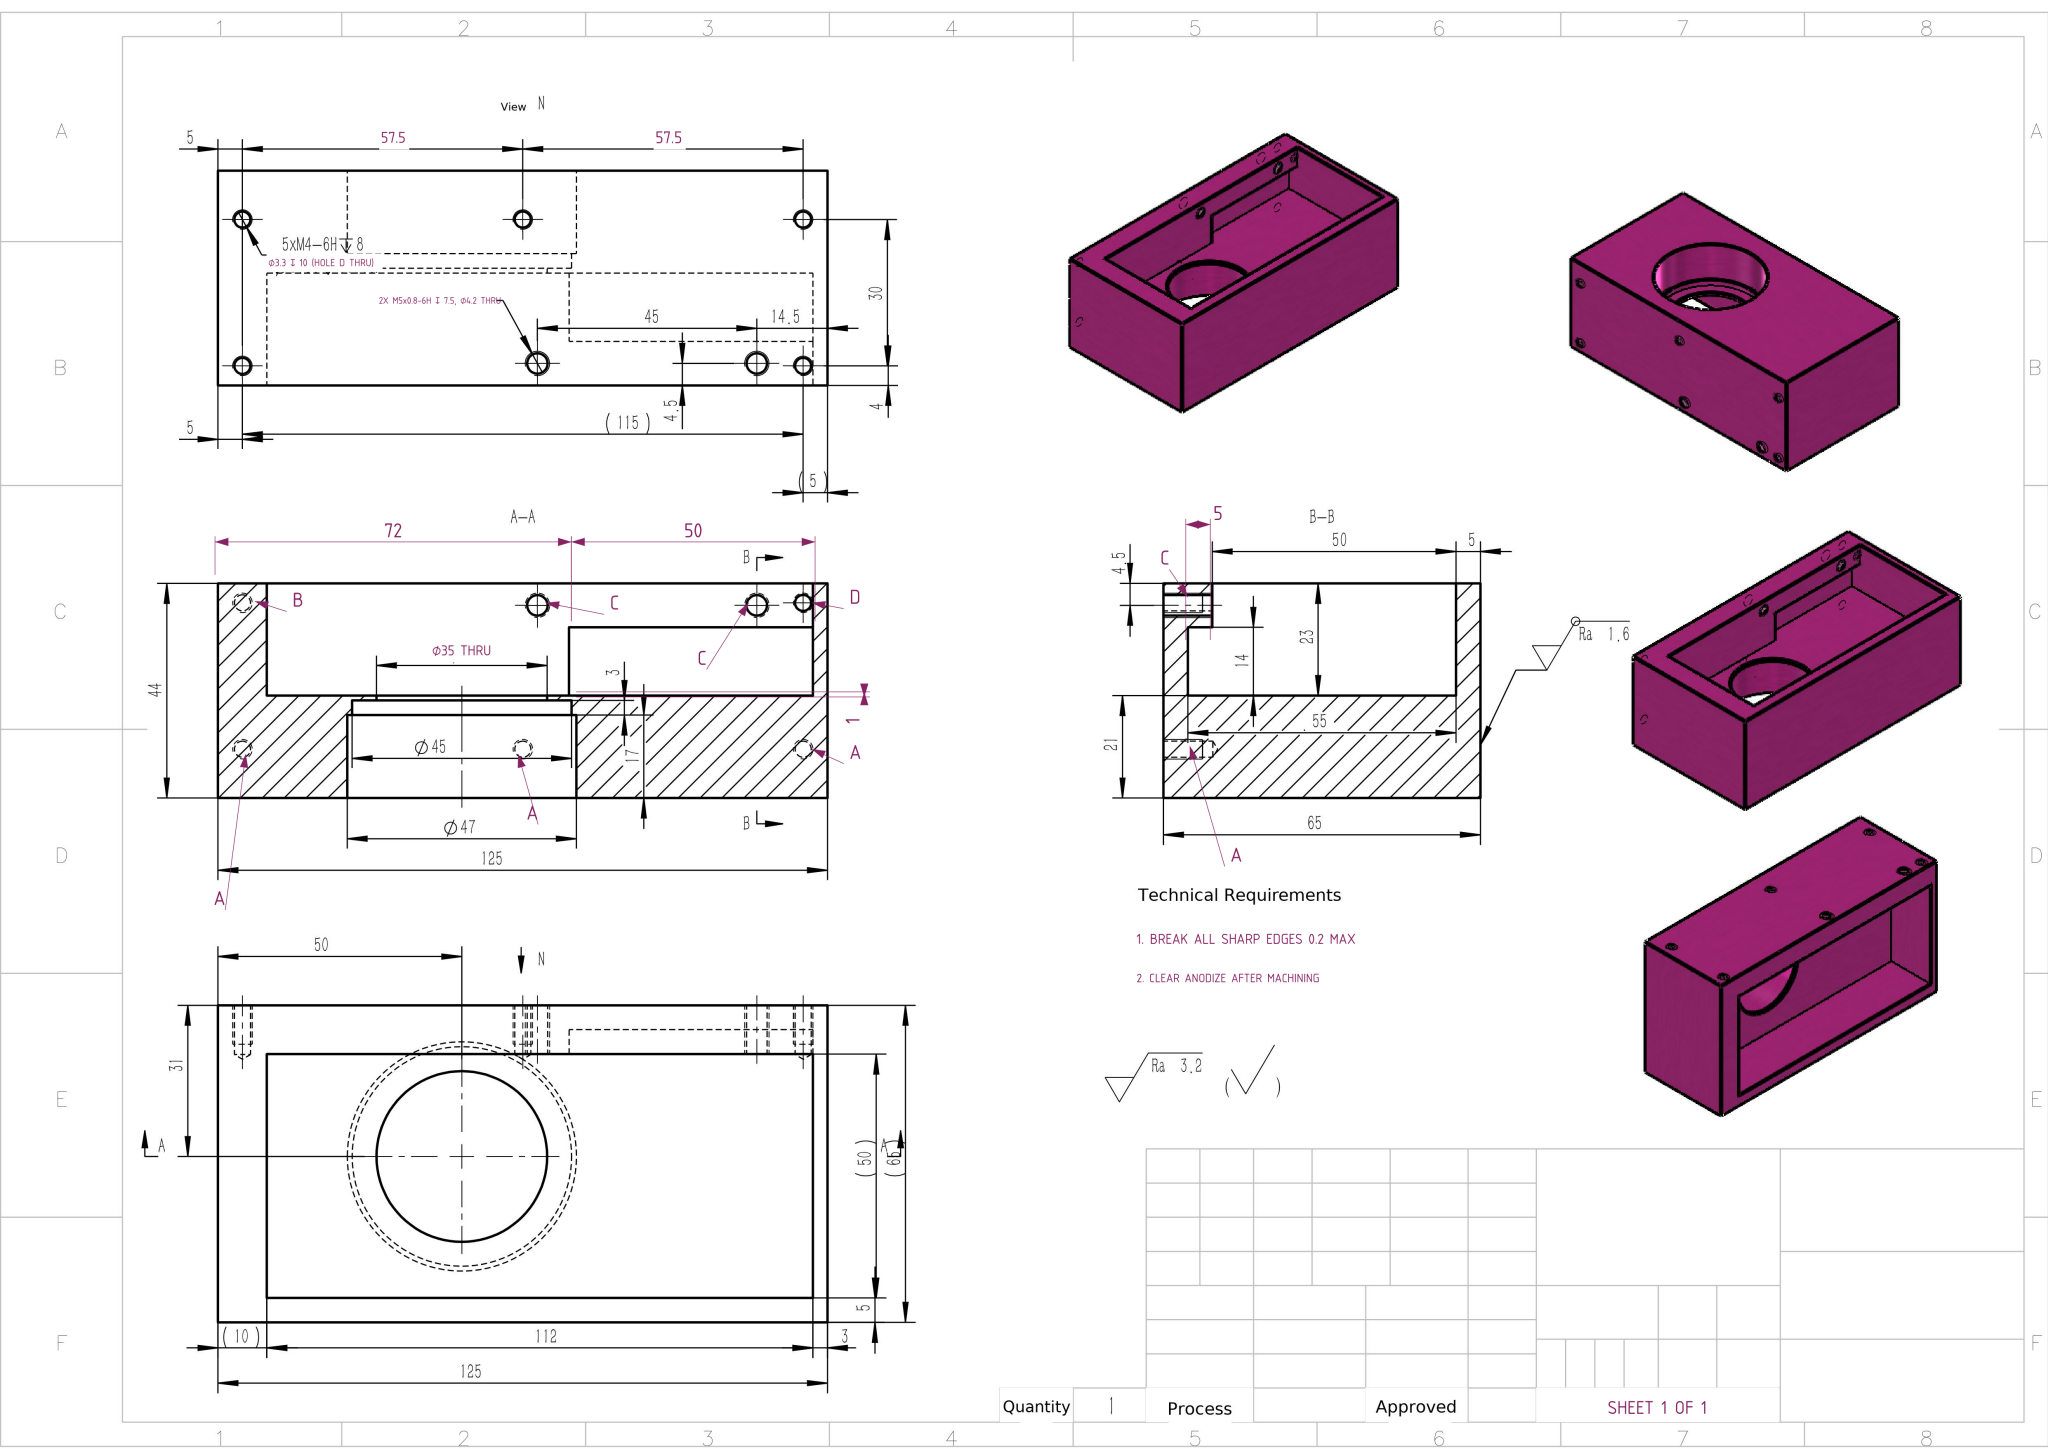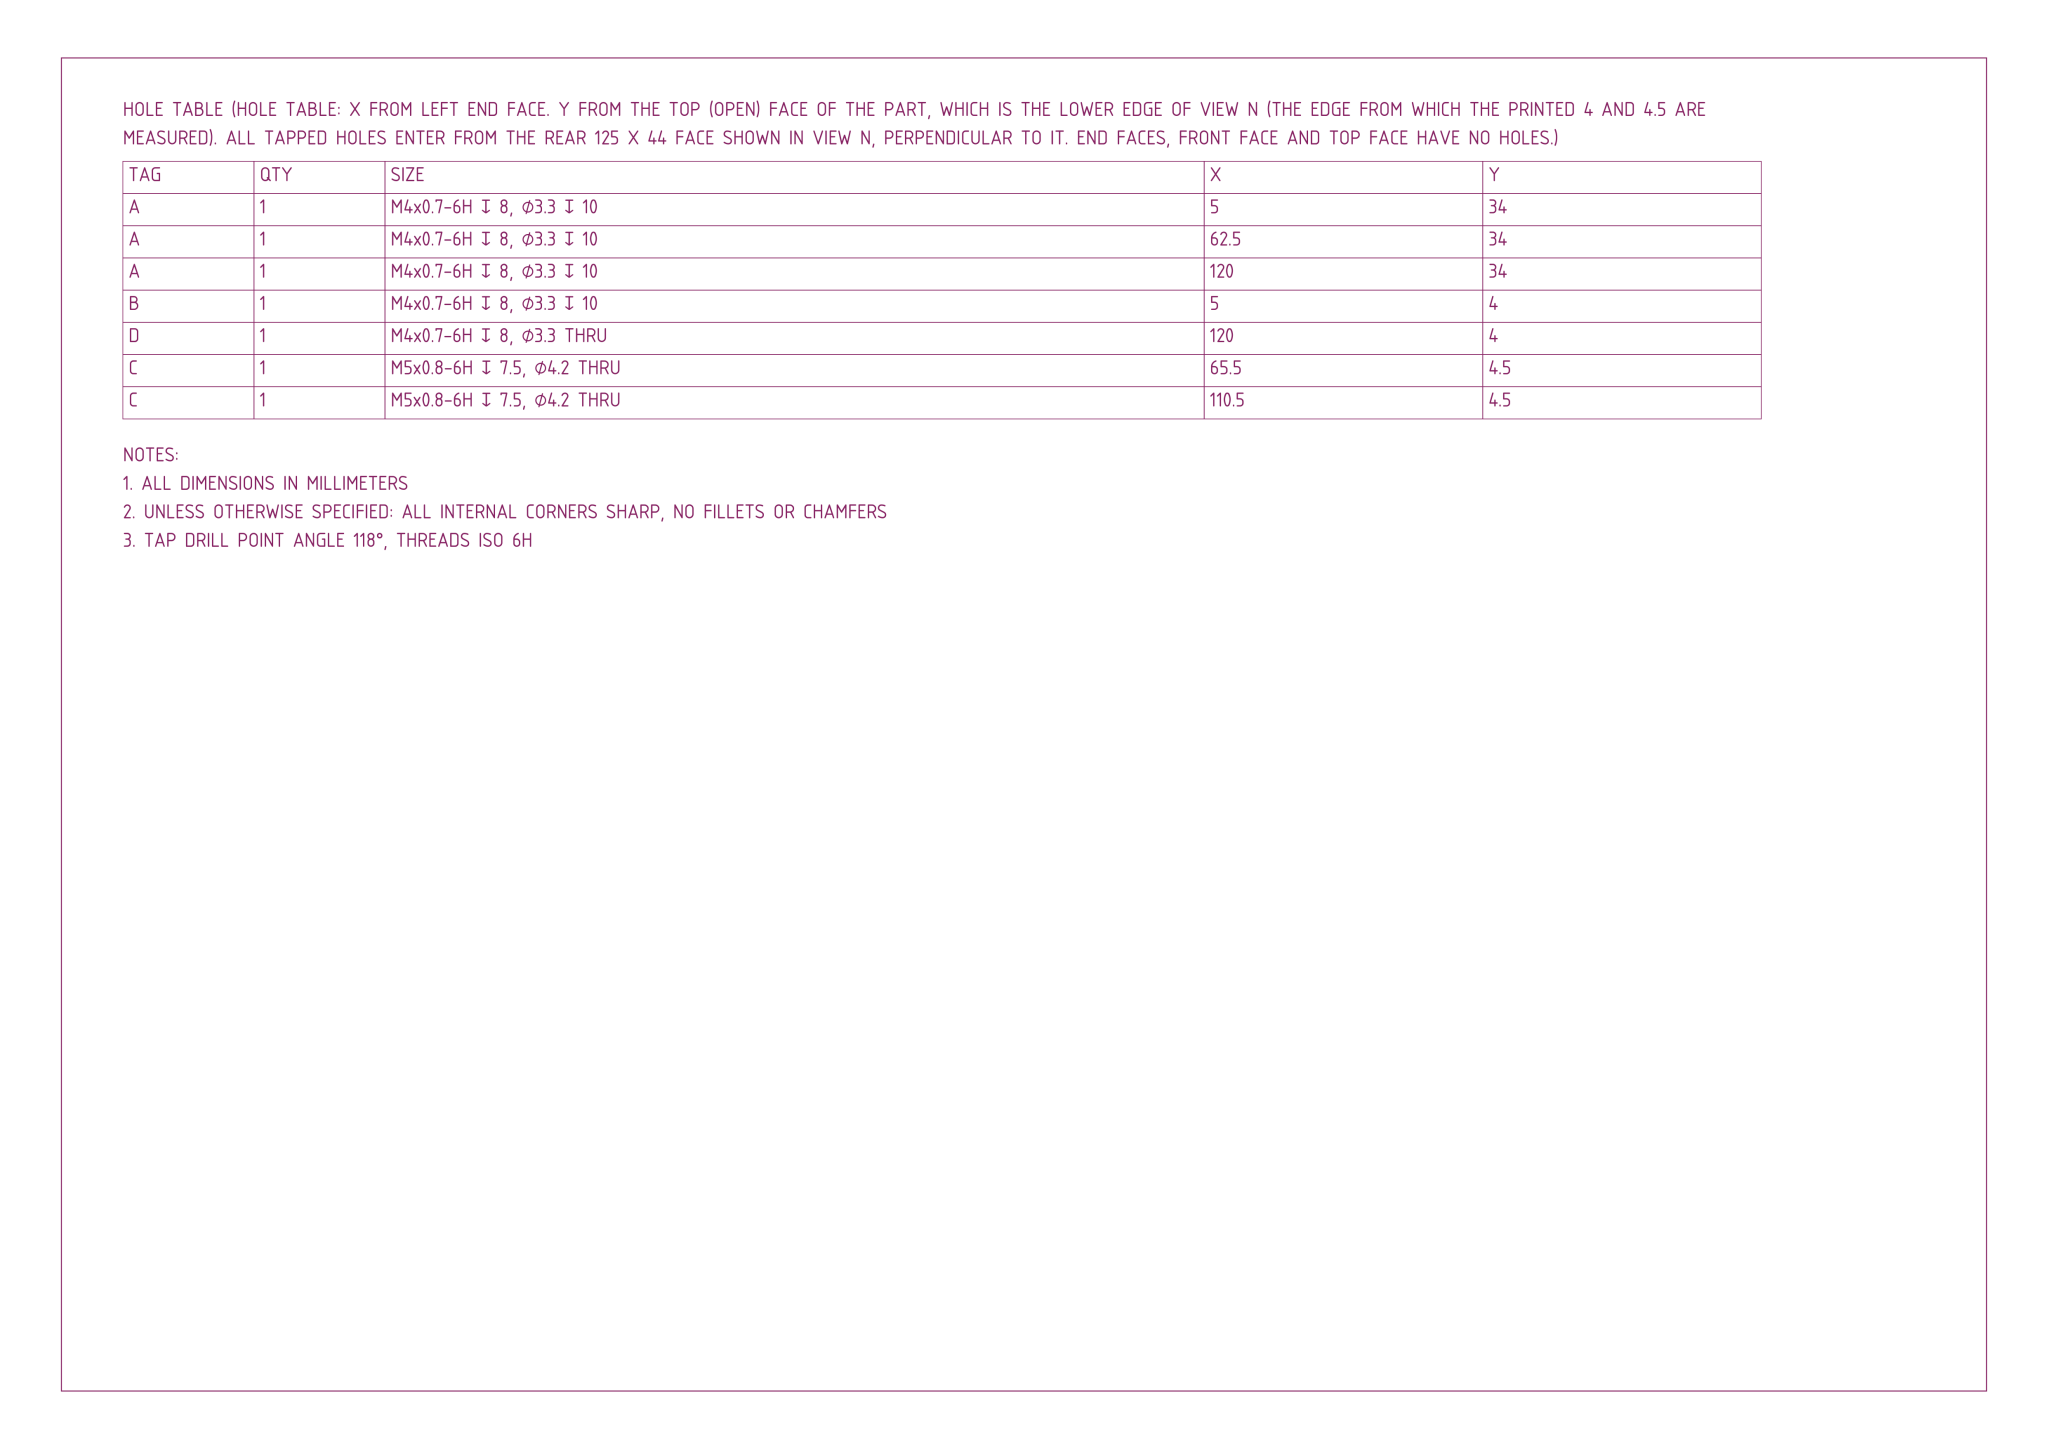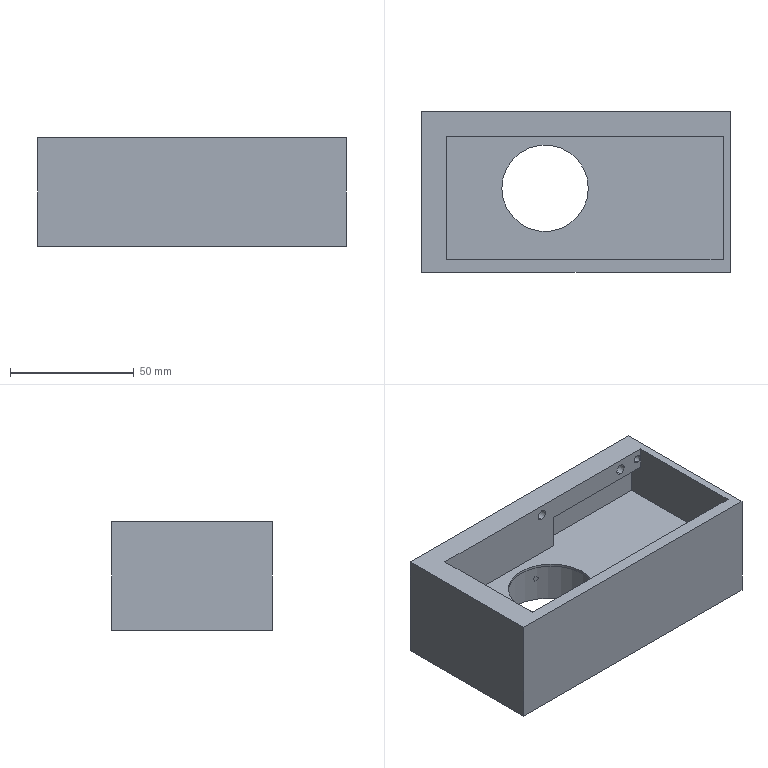Part | NX | mm | 1 solid | 44 faces | box 125 x 65 x 44 mm | volume 189253 mm3 | cylinder 20 | plane 16 | cone 8 | commonest cylinder face diameters 3.3 x10 4.2 x4 47 x2 35 x2 45 x2